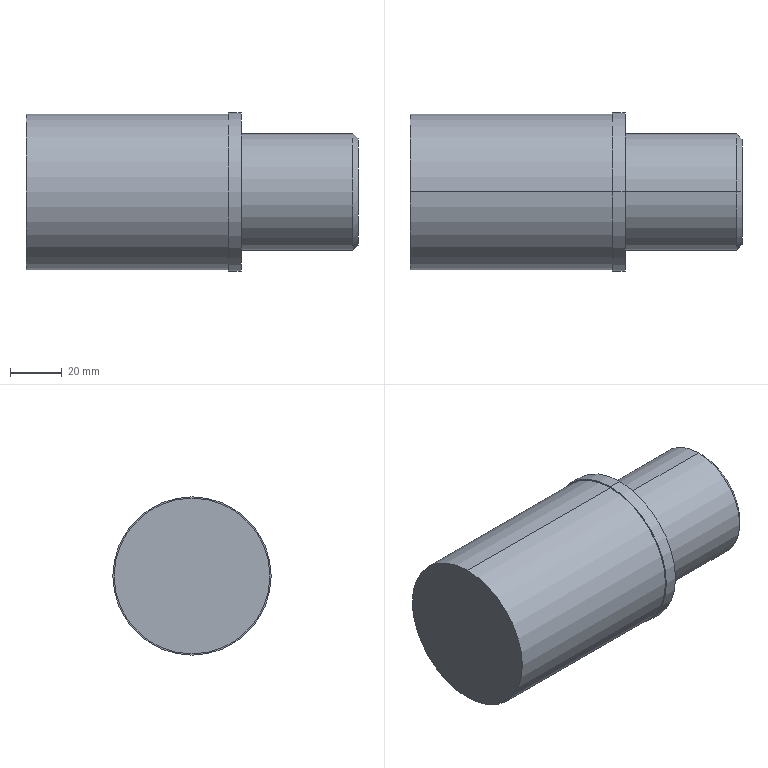Component | SolidWorks | YC1-250-03-01SliderAssembly-1_YC1-250-03-27BalancerConnectingPin-1 | 1 solid | 16 faces | box 128 x 61 x 61 mm | volume 305264 mm3 | cylinder 8 | cone 4 | plane 4 | commonest cylinder face diameters 60 x2 61 x2 45 x2 8.5 x2 | material Plain Carbon Steel
STEP:
#1=COLOUR_RGB('',0.7922,0.8196,0.9333);
#2=FILL_AREA_STYLE_COLOUR('',#1);
#3=FILL_AREA_STYLE('',(#2));
#4=SURFACE_STYLE_FILL_AREA(#3);
#5=SURFACE_SIDE_STYLE('',(#4));
#6=SURFACE_STYLE_USAGE(.BOTH.,#5);
#7=PRESENTATION_STYLE_ASSIGNMENT((#6));
#8=CARTESIAN_POINT('',(-16.732,110.632,1.181));
#9=VERTEX_POINT('',#8);
#10=CARTESIAN_POINT('',(-16.732,110.632,-1.181));
#11=VERTEX_POINT('',#10);
#12=CARTESIAN_POINT('',(-16.732,110.632,-0.));
#13=DIRECTION('',(-1.,0.,0.));
#14=DIRECTION('',(0.,0.,1.));
#15=AXIS2_PLACEMENT_3D('',#12,#13,#14);
#16=CIRCLE('',#15,1.181);
#17=EDGE_CURVE('',#9,#11,#16,.T.);
#18=ORIENTED_EDGE('',*,*,#17,.T.);
#19=CARTESIAN_POINT('',(-19.803,110.632,-1.181));
#20=VERTEX_POINT('',#19);
#21=CARTESIAN_POINT('',(-19.803,110.632,-1.181));
#22=DIRECTION('',(-1.,0.,0.));
#23=VECTOR('',#22,39.37);
#24=LINE('',#21,#23);
#25=EDGE_CURVE('',#11,#20,#24,.T.);
#26=ORIENTED_EDGE('',*,*,#25,.T.);
#27=CARTESIAN_POINT('',(-19.803,110.632,1.181));
#28=VERTEX_POINT('',#27);
#29=CARTESIAN_POINT('',(-19.803,110.632,-0.));
#30=DIRECTION('',(1.,0.,0.));
#31=DIRECTION('',(0.,0.,1.));
#32=AXIS2_PLACEMENT_3D('',#29,#30,#31);
#33=CIRCLE('',#32,1.181);
#34=EDGE_CURVE('',#20,#28,#33,.T.);
#35=ORIENTED_EDGE('',*,*,#34,.T.);
#36=CARTESIAN_POINT('',(-19.803,110.632,1.181));
#37=DIRECTION('',(-1.,0.,0.));
#38=VECTOR('',#37,39.37);
#39=LINE('',#36,#38);
#40=EDGE_CURVE('',#9,#28,#39,.T.);
#41=ORIENTED_EDGE('',*,*,#40,.F.);
#42=EDGE_LOOP('',(#18,#26,#35,#41));
#43=FACE_OUTER_BOUND('',#42,.T.);
#44=CARTESIAN_POINT('',(-19.803,110.632,-0.));
#45=DIRECTION('',(-1.,0.,0.));
#46=DIRECTION('',(0.,0.,1.));
#47=AXIS2_PLACEMENT_3D('',#44,#45,#46);
#48=CYLINDRICAL_SURFACE('',#47,1.181);
#49=ADVANCED_FACE('',(#43),#48,.T.);
#50=CARTESIAN_POINT('',(-16.535,110.632,1.201));
#51=VERTEX_POINT('',#50);
#52=CARTESIAN_POINT('',(-16.535,110.632,-1.201));
#53=VERTEX_POINT('',#52);
#54=CARTESIAN_POINT('',(-16.535,110.632,-0.));
#55=DIRECTION('',(-1.,0.,0.));
#56=DIRECTION('',(0.,0.,1.));
#57=AXIS2_PLACEMENT_3D('',#54,#55,#56);
#58=CIRCLE('',#57,1.201);
#59=EDGE_CURVE('',#51,#53,#58,.T.);
#60=ORIENTED_EDGE('',*,*,#59,.T.);
#61=CARTESIAN_POINT('',(-16.732,110.632,-1.201));
#62=VERTEX_POINT('',#61);
#63=CARTESIAN_POINT('',(-19.803,110.632,-1.201));
#64=DIRECTION('',(-1.,0.,0.));
#65=VECTOR('',#64,39.37);
#66=LINE('',#63,#65);
#67=EDGE_CURVE('',#53,#62,#66,.T.);
#68=ORIENTED_EDGE('',*,*,#67,.T.);
#69=CARTESIAN_POINT('',(-16.732,110.632,1.201));
#70=VERTEX_POINT('',#69);
#71=CARTESIAN_POINT('',(-16.732,110.632,-0.));
#72=DIRECTION('',(1.,0.,0.));
#73=DIRECTION('',(0.,0.,1.));
#74=AXIS2_PLACEMENT_3D('',#71,#72,#73);
#75=CIRCLE('',#74,1.201);
#76=EDGE_CURVE('',#62,#70,#75,.T.);
#77=ORIENTED_EDGE('',*,*,#76,.T.);
#78=CARTESIAN_POINT('',(-19.803,110.632,1.201));
#79=DIRECTION('',(-1.,0.,0.));
#80=VECTOR('',#79,39.37);
#81=LINE('',#78,#80);
#82=EDGE_CURVE('',#51,#70,#81,.T.);
#83=ORIENTED_EDGE('',*,*,#82,.F.);
#84=EDGE_LOOP('',(#60,#68,#77,#83));
#85=FACE_OUTER_BOUND('',#84,.T.);
#86=CARTESIAN_POINT('',(-19.803,110.632,-0.));
#87=DIRECTION('',(-1.,0.,0.));
#88=DIRECTION('',(0.,0.,1.));
#89=AXIS2_PLACEMENT_3D('',#86,#87,#88);
#90=CYLINDRICAL_SURFACE('',#89,1.201);
#91=ADVANCED_FACE('',(#85),#90,.T.);
#92=CARTESIAN_POINT('',(-14.843,110.632,0.8858));
#93=VERTEX_POINT('',#92);
#94=CARTESIAN_POINT('',(-14.843,110.632,-0.8858));
#95=VERTEX_POINT('',#94);
#96=CARTESIAN_POINT('',(-14.843,110.632,-0.));
#97=DIRECTION('',(-1.,0.,0.));
#98=DIRECTION('',(0.,0.,1.));
#99=AXIS2_PLACEMENT_3D('',#96,#97,#98);
#100=CIRCLE('',#99,0.8858);
#101=EDGE_CURVE('',#93,#95,#100,.T.);
#102=ORIENTED_EDGE('',*,*,#101,.T.);
#103=CARTESIAN_POINT('',(-16.535,110.632,-0.8858));
#104=VERTEX_POINT('',#103);
#105=CARTESIAN_POINT('',(-19.803,110.632,-0.8858));
#106=DIRECTION('',(-1.,0.,0.));
#107=VECTOR('',#106,39.37);
#108=LINE('',#105,#107);
#109=EDGE_CURVE('',#95,#104,#108,.T.);
#110=ORIENTED_EDGE('',*,*,#109,.T.);
#111=CARTESIAN_POINT('',(-16.535,110.632,0.8858));
#112=VERTEX_POINT('',#111);
#113=CARTESIAN_POINT('',(-16.535,110.632,-0.));
#114=DIRECTION('',(1.,0.,0.));
#115=DIRECTION('',(0.,0.,1.));
#116=AXIS2_PLACEMENT_3D('',#113,#114,#115);
#117=CIRCLE('',#116,0.8858);
#118=EDGE_CURVE('',#104,#112,#117,.T.);
#119=ORIENTED_EDGE('',*,*,#118,.T.);
#120=CARTESIAN_POINT('',(-19.803,110.632,0.8858));
#121=DIRECTION('',(-1.,0.,0.));
#122=VECTOR('',#121,39.37);
#123=LINE('',#120,#122);
#124=EDGE_CURVE('',#93,#112,#123,.T.);
#125=ORIENTED_EDGE('',*,*,#124,.F.);
#126=EDGE_LOOP('',(#102,#110,#119,#125));
#127=FACE_OUTER_BOUND('',#126,.T.);
#128=CARTESIAN_POINT('',(-19.803,110.632,-0.));
#129=DIRECTION('',(-1.,0.,0.));
#130=DIRECTION('',(0.,0.,1.));
#131=AXIS2_PLACEMENT_3D('',#128,#129,#130);
#132=CYLINDRICAL_SURFACE('',#131,0.8858);
#133=ADVANCED_FACE('',(#127),#132,.T.);
#134=CARTESIAN_POINT('',(-14.764,110.632,0.8071));
#135=VERTEX_POINT('',#134);
#136=CARTESIAN_POINT('',(-14.764,110.632,-0.8071));
#137=VERTEX_POINT('',#136);
#138=CARTESIAN_POINT('',(-14.764,110.632,-0.));
#139=DIRECTION('',(-1.,0.,0.));
#140=DIRECTION('',(0.,0.,1.));
#141=AXIS2_PLACEMENT_3D('',#138,#139,#140);
#142=CIRCLE('',#141,0.8071);
#143=EDGE_CURVE('',#135,#137,#142,.T.);
#144=ORIENTED_EDGE('',*,*,#143,.T.);
#145=CARTESIAN_POINT('',(-14.843,110.632,-0.8858));
#146=DIRECTION('',(-0.7071,0.,-0.7071));
#147=VECTOR('',#146,39.37);
#148=LINE('',#145,#147);
#149=EDGE_CURVE('',#137,#95,#148,.T.);
#150=ORIENTED_EDGE('',*,*,#149,.T.);
#151=ORIENTED_EDGE('',*,*,#101,.F.);
#152=CARTESIAN_POINT('',(-14.843,110.632,0.8858));
#153=DIRECTION('',(-0.7071,0.,0.7071));
#154=VECTOR('',#153,39.37);
#155=LINE('',#152,#154);
#156=EDGE_CURVE('',#135,#93,#155,.T.);
#157=ORIENTED_EDGE('',*,*,#156,.F.);
#158=EDGE_LOOP('',(#144,#150,#151,#157));
#159=FACE_OUTER_BOUND('',#158,.T.);
#160=CARTESIAN_POINT('',(-14.843,110.632,-0.));
#161=DIRECTION('',(-1.,0.,0.));
#162=DIRECTION('',(0.,0.,1.));
#163=AXIS2_PLACEMENT_3D('',#160,#161,#162);
#164=CONICAL_SURFACE('',#163,0.8858,0.7854);
#165=ADVANCED_FACE('',(#159),#164,.T.);
#166=CARTESIAN_POINT('',(-15.551,110.632,0.1673));
#167=VERTEX_POINT('',#166);
#168=CARTESIAN_POINT('',(-15.551,110.632,-0.1673));
#169=VERTEX_POINT('',#168);
#170=CARTESIAN_POINT('',(-15.551,110.632,-0.));
#171=DIRECTION('',(1.,0.,0.));
#172=DIRECTION('',(0.,0.,-1.));
#173=AXIS2_PLACEMENT_3D('',#170,#171,#172);
#174=CIRCLE('',#173,0.1673);
#175=EDGE_CURVE('',#167,#169,#174,.T.);
#176=ORIENTED_EDGE('',*,*,#175,.F.);
#177=CARTESIAN_POINT('',(-14.764,110.632,0.1673));
#178=VERTEX_POINT('',#177);
#179=CARTESIAN_POINT('',(-14.764,110.632,0.1673));
#180=DIRECTION('',(1.,0.,0.));
#181=VECTOR('',#180,39.37);
#182=LINE('',#179,#181);
#183=EDGE_CURVE('',#167,#178,#182,.T.);
#184=ORIENTED_EDGE('',*,*,#183,.T.);
#185=CARTESIAN_POINT('',(-14.764,110.632,-0.1673));
#186=VERTEX_POINT('',#185);
#187=CARTESIAN_POINT('',(-14.764,110.632,-0.));
#188=DIRECTION('',(1.,0.,0.));
#189=DIRECTION('',(0.,0.,-1.));
#190=AXIS2_PLACEMENT_3D('',#187,#188,#189);
#191=CIRCLE('',#190,0.1673);
#192=EDGE_CURVE('',#178,#186,#191,.T.);
#193=ORIENTED_EDGE('',*,*,#192,.T.);
#194=CARTESIAN_POINT('',(-14.764,110.632,-0.1673));
#195=DIRECTION('',(1.,0.,0.));
#196=VECTOR('',#195,39.37);
#197=LINE('',#194,#196);
#198=EDGE_CURVE('',#169,#186,#197,.T.);
#199=ORIENTED_EDGE('',*,*,#198,.F.);
#200=EDGE_LOOP('',(#176,#184,#193,#199));
#201=FACE_OUTER_BOUND('',#200,.T.);
#202=CARTESIAN_POINT('',(-14.764,110.632,-0.));
#203=DIRECTION('',(1.,0.,0.));
#204=DIRECTION('',(0.,0.,-1.));
#205=AXIS2_PLACEMENT_3D('',#202,#203,#204);
#206=CYLINDRICAL_SURFACE('',#205,0.1673);
#207=ADVANCED_FACE('',(#201),#206,.F.);
#208=CARTESIAN_POINT('',(-15.652,110.632,-0.));
#209=VERTEX_POINT('',#208);
#210=CARTESIAN_POINT('',(-15.551,110.632,-0.1673));
#211=DIRECTION('',(0.515,0.,-0.8572));
#212=VECTOR('',#211,39.37);
#213=LINE('',#210,#212);
#214=EDGE_CURVE('',#209,#169,#213,.T.);
#215=ORIENTED_EDGE('',*,*,#214,.F.);
#216=CARTESIAN_POINT('',(-15.551,110.632,0.1673));
#217=DIRECTION('',(0.515,0.,0.8572));
#218=VECTOR('',#217,39.37);
#219=LINE('',#216,#218);
#220=EDGE_CURVE('',#209,#167,#219,.T.);
#221=ORIENTED_EDGE('',*,*,#220,.T.);
#222=ORIENTED_EDGE('',*,*,#175,.T.);
#223=EDGE_LOOP('',(#215,#221,#222));
#224=FACE_OUTER_BOUND('',#223,.T.);
#225=CARTESIAN_POINT('',(-15.551,110.632,-0.));
#226=DIRECTION('',(1.,0.,0.));
#227=DIRECTION('',(0.,0.,-1.));
#228=AXIS2_PLACEMENT_3D('',#225,#226,#227);
#229=CONICAL_SURFACE('',#228,0.1673,1.03);
#230=ADVANCED_FACE('',(#224),#229,.F.);
#231=ORIENTED_EDGE('',*,*,#25,.F.);
#232=CARTESIAN_POINT('',(-16.732,110.632,-0.));
#233=DIRECTION('',(-1.,0.,0.));
#234=DIRECTION('',(0.,0.,1.));
#235=AXIS2_PLACEMENT_3D('',#232,#233,#234);
#236=CIRCLE('',#235,1.181);
#237=EDGE_CURVE('',#11,#9,#236,.T.);
#238=ORIENTED_EDGE('',*,*,#237,.T.);
#239=ORIENTED_EDGE('',*,*,#40,.T.);
#240=CARTESIAN_POINT('',(-19.803,110.632,-0.));
#241=DIRECTION('',(1.,0.,0.));
#242=DIRECTION('',(0.,0.,1.));
#243=AXIS2_PLACEMENT_3D('',#240,#241,#242);
#244=CIRCLE('',#243,1.181);
#245=EDGE_CURVE('',#28,#20,#244,.T.);
#246=ORIENTED_EDGE('',*,*,#245,.T.);
#247=EDGE_LOOP('',(#231,#238,#239,#246));
#248=FACE_OUTER_BOUND('',#247,.T.);
#249=CARTESIAN_POINT('',(-19.803,110.632,-0.));
#250=DIRECTION('',(-1.,0.,0.));
#251=DIRECTION('',(0.,0.,1.));
#252=AXIS2_PLACEMENT_3D('',#249,#250,#251);
#253=CYLINDRICAL_SURFACE('',#252,1.181);
#254=ADVANCED_FACE('',(#248),#253,.T.);
#255=ORIENTED_EDGE('',*,*,#245,.F.);
#256=ORIENTED_EDGE('',*,*,#34,.F.);
#257=EDGE_LOOP('',(#255,#256));
#258=FACE_OUTER_BOUND('',#257,.T.);
#259=CARTESIAN_POINT('',(-19.803,110.632,-0.));
#260=DIRECTION('',(1.,0.,0.));
#261=DIRECTION('',(0.,0.,-1.));
#262=AXIS2_PLACEMENT_3D('',#259,#260,#261);
#263=PLANE('',#262);
#264=ADVANCED_FACE('',(#258),#263,.F.);
#265=CARTESIAN_POINT('',(-16.732,110.632,-0.));
#266=DIRECTION('',(1.,0.,0.));
#267=DIRECTION('',(0.,0.,1.));
#268=AXIS2_PLACEMENT_3D('',#265,#266,#267);
#269=CIRCLE('',#268,1.201);
#270=EDGE_CURVE('',#70,#62,#269,.T.);
#271=ORIENTED_EDGE('',*,*,#270,.F.);
#272=ORIENTED_EDGE('',*,*,#76,.F.);
#273=EDGE_LOOP('',(#271,#272));
#274=FACE_OUTER_BOUND('',#273,.T.);
#275=ORIENTED_EDGE('',*,*,#17,.F.);
#276=ORIENTED_EDGE('',*,*,#237,.F.);
#277=EDGE_LOOP('',(#275,#276));
#278=FACE_BOUND('',#277,.T.);
#279=CARTESIAN_POINT('',(-16.732,111.813,-0.));
#280=DIRECTION('',(1.,0.,0.));
#281=DIRECTION('',(0.,0.,-1.));
#282=AXIS2_PLACEMENT_3D('',#279,#280,#281);
#283=PLANE('',#282);
#284=ADVANCED_FACE('',(#274,#278),#283,.F.);
#285=ORIENTED_EDGE('',*,*,#67,.F.);
#286=CARTESIAN_POINT('',(-16.535,110.632,-0.));
#287=DIRECTION('',(-1.,0.,0.));
#288=DIRECTION('',(0.,0.,1.));
#289=AXIS2_PLACEMENT_3D('',#286,#287,#288);
#290=CIRCLE('',#289,1.201);
#291=EDGE_CURVE('',#53,#51,#290,.T.);
#292=ORIENTED_EDGE('',*,*,#291,.T.);
#293=ORIENTED_EDGE('',*,*,#82,.T.);
#294=ORIENTED_EDGE('',*,*,#270,.T.);
#295=EDGE_LOOP('',(#285,#292,#293,#294));
#296=FACE_OUTER_BOUND('',#295,.T.);
#297=CARTESIAN_POINT('',(-19.803,110.632,-0.));
#298=DIRECTION('',(-1.,0.,0.));
#299=DIRECTION('',(0.,0.,1.));
#300=AXIS2_PLACEMENT_3D('',#297,#298,#299);
#301=CYLINDRICAL_SURFACE('',#300,1.201);
#302=ADVANCED_FACE('',(#296),#301,.T.);
#303=CARTESIAN_POINT('',(-16.535,110.632,-0.));
#304=DIRECTION('',(1.,0.,0.));
#305=DIRECTION('',(0.,0.,1.));
#306=AXIS2_PLACEMENT_3D('',#303,#304,#305);
#307=CIRCLE('',#306,0.8858);
#308=EDGE_CURVE('',#112,#104,#307,.T.);
#309=ORIENTED_EDGE('',*,*,#308,.F.);
#310=ORIENTED_EDGE('',*,*,#118,.F.);
#311=EDGE_LOOP('',(#309,#310));
#312=FACE_BOUND('',#311,.T.);
#313=ORIENTED_EDGE('',*,*,#59,.F.);
#314=ORIENTED_EDGE('',*,*,#291,.F.);
#315=EDGE_LOOP('',(#313,#314));
#316=FACE_OUTER_BOUND('',#315,.T.);
#317=CARTESIAN_POINT('',(-16.535,111.833,-0.));
#318=DIRECTION('',(-1.,0.,0.));
#319=DIRECTION('',(0.,0.,1.));
#320=AXIS2_PLACEMENT_3D('',#317,#318,#319);
#321=PLANE('',#320);
#322=ADVANCED_FACE('',(#312,#316),#321,.F.);
#323=ORIENTED_EDGE('',*,*,#109,.F.);
#324=CARTESIAN_POINT('',(-14.843,110.632,-0.));
#325=DIRECTION('',(-1.,0.,0.));
#326=DIRECTION('',(0.,0.,1.));
#327=AXIS2_PLACEMENT_3D('',#324,#325,#326);
#328=CIRCLE('',#327,0.8858);
#329=EDGE_CURVE('',#95,#93,#328,.T.);
#330=ORIENTED_EDGE('',*,*,#329,.T.);
#331=ORIENTED_EDGE('',*,*,#124,.T.);
#332=ORIENTED_EDGE('',*,*,#308,.T.);
#333=EDGE_LOOP('',(#323,#330,#331,#332));
#334=FACE_OUTER_BOUND('',#333,.T.);
#335=CARTESIAN_POINT('',(-19.803,110.632,-0.));
#336=DIRECTION('',(-1.,0.,0.));
#337=DIRECTION('',(0.,0.,1.));
#338=AXIS2_PLACEMENT_3D('',#335,#336,#337);
#339=CYLINDRICAL_SURFACE('',#338,0.8858);
#340=ADVANCED_FACE('',(#334),#339,.T.);
#341=ORIENTED_EDGE('',*,*,#149,.F.);
#342=CARTESIAN_POINT('',(-14.764,110.632,-0.));
#343=DIRECTION('',(-1.,0.,0.));
#344=DIRECTION('',(0.,0.,1.));
#345=AXIS2_PLACEMENT_3D('',#342,#343,#344);
#346=CIRCLE('',#345,0.8071);
#347=EDGE_CURVE('',#137,#135,#346,.T.);
#348=ORIENTED_EDGE('',*,*,#347,.T.);
#349=ORIENTED_EDGE('',*,*,#156,.T.);
#350=ORIENTED_EDGE('',*,*,#329,.F.);
#351=EDGE_LOOP('',(#341,#348,#349,#350));
#352=FACE_OUTER_BOUND('',#351,.T.);
#353=CARTESIAN_POINT('',(-14.843,110.632,-0.));
#354=DIRECTION('',(-1.,0.,0.));
#355=DIRECTION('',(0.,0.,1.));
#356=AXIS2_PLACEMENT_3D('',#353,#354,#355);
#357=CONICAL_SURFACE('',#356,0.8858,0.7854);
#358=ADVANCED_FACE('',(#352),#357,.T.);
#359=ORIENTED_EDGE('',*,*,#143,.F.);
#360=ORIENTED_EDGE('',*,*,#347,.F.);
#361=EDGE_LOOP('',(#359,#360));
#362=FACE_OUTER_BOUND('',#361,.T.);
#363=CARTESIAN_POINT('',(-14.764,110.632,-0.));
#364=DIRECTION('',(1.,0.,0.));
#365=DIRECTION('',(0.,0.,-1.));
#366=AXIS2_PLACEMENT_3D('',#363,#364,#365);
#367=CIRCLE('',#366,0.1673);
#368=EDGE_CURVE('',#186,#178,#367,.T.);
#369=ORIENTED_EDGE('',*,*,#368,.F.);
#370=ORIENTED_EDGE('',*,*,#192,.F.);
#371=EDGE_LOOP('',(#369,#370));
#372=FACE_BOUND('',#371,.T.);
#373=CARTESIAN_POINT('',(-14.764,111.518,-0.));
#374=DIRECTION('',(-1.,0.,0.));
#375=DIRECTION('',(0.,0.,1.));
#376=AXIS2_PLACEMENT_3D('',#373,#374,#375);
#377=PLANE('',#376);
#378=ADVANCED_FACE('',(#362,#372),#377,.F.);
#379=ORIENTED_EDGE('',*,*,#183,.F.);
#380=CARTESIAN_POINT('',(-15.551,110.632,-0.));
#381=DIRECTION('',(1.,0.,0.));
#382=DIRECTION('',(0.,0.,-1.));
#383=AXIS2_PLACEMENT_3D('',#380,#381,#382);
#384=CIRCLE('',#383,0.1673);
#385=EDGE_CURVE('',#169,#167,#384,.T.);
#386=ORIENTED_EDGE('',*,*,#385,.F.);
#387=ORIENTED_EDGE('',*,*,#198,.T.);
#388=ORIENTED_EDGE('',*,*,#368,.T.);
#389=EDGE_LOOP('',(#379,#386,#387,#388));
#390=FACE_OUTER_BOUND('',#389,.T.);
#391=CARTESIAN_POINT('',(-14.764,110.632,-0.));
#392=DIRECTION('',(1.,0.,0.));
#393=DIRECTION('',(0.,0.,-1.));
#394=AXIS2_PLACEMENT_3D('',#391,#392,#393);
#395=CYLINDRICAL_SURFACE('',#394,0.1673);
#396=ADVANCED_FACE('',(#390),#395,.F.);
#397=ORIENTED_EDGE('',*,*,#220,.F.);
#398=ORIENTED_EDGE('',*,*,#214,.T.);
#399=ORIENTED_EDGE('',*,*,#385,.T.);
#400=EDGE_LOOP('',(#397,#398,#399));
#401=FACE_OUTER_BOUND('',#400,.T.);
#402=CARTESIAN_POINT('',(-15.551,110.632,-0.));
#403=DIRECTION('',(1.,0.,0.));
#404=DIRECTION('',(0.,0.,-1.));
#405=AXIS2_PLACEMENT_3D('',#402,#403,#404);
#406=CONICAL_SURFACE('',#405,0.1673,1.03);
#407=ADVANCED_FACE('',(#401),#406,.F.);
#408=CLOSED_SHELL('',(#49,#91,#133,#165,#207,#230,#254,#264,#284,#302,#322,#340,#358,#378,#396,#407));
#409=MANIFOLD_SOLID_BREP('',#408);
#410=STYLED_ITEM('',(#7),#409);
#411=(LENGTH_UNIT()NAMED_UNIT(*)SI_UNIT($,.METRE.));
#412=LENGTH_MEASURE_WITH_UNIT(LENGTH_MEASURE(0.0254),#411);
#413=DIMENSIONAL_EXPONENTS(1.,0.,0.,0.,0.,0.,0.);
#414=(CONVERSION_BASED_UNIT('',#412)LENGTH_UNIT()NAMED_UNIT(#413));
#415=UNCERTAINTY_MEASURE_WITH_UNIT(LENGTH_MEASURE(0.00001),#414,'','');
#416=(NAMED_UNIT(*)PLANE_ANGLE_UNIT()SI_UNIT($,.RADIAN.));
#417=(NAMED_UNIT(*)SI_UNIT($,.STERADIAN.)SOLID_ANGLE_UNIT());
#418=(GEOMETRIC_REPRESENTATION_CONTEXT(3)GLOBAL_UNCERTAINTY_ASSIGNED_CONTEXT((#415))GLOBAL_UNIT_ASSIGNED_CONTEXT((#414,#416,#417))REPRESENTATION_CONTEXT('',''));
#419=MECHANICAL_DESIGN_GEOMETRIC_PRESENTATION_REPRESENTATION('',(#410),#418);
#420=CARTESIAN_POINT('',(0.,0.,0.));
#421=DIRECTION('',(0.,0.,1.));
#422=DIRECTION('',(1.,0.,0.));
#423=AXIS2_PLACEMENT_3D('',#420,#421,#422);
#424=(LENGTH_UNIT()NAMED_UNIT(*)SI_UNIT($,.METRE.));
#425=LENGTH_MEASURE_WITH_UNIT(LENGTH_MEASURE(0.0254),#424);
#426=DIMENSIONAL_EXPONENTS(1.,0.,0.,0.,0.,0.,0.);
#427=(CONVERSION_BASED_UNIT('',#425)LENGTH_UNIT()NAMED_UNIT(#426));
#428=UNCERTAINTY_MEASURE_WITH_UNIT(LENGTH_MEASURE(0.00001),#427,'','');
#429=(NAMED_UNIT(*)PLANE_ANGLE_UNIT()SI_UNIT($,.RADIAN.));
#430=(NAMED_UNIT(*)SI_UNIT($,.STERADIAN.)SOLID_ANGLE_UNIT());
#431=(GEOMETRIC_REPRESENTATION_CONTEXT(3)GLOBAL_UNCERTAINTY_ASSIGNED_CONTEXT((#428))GLOBAL_UNIT_ASSIGNED_CONTEXT((#427,#429,#430))REPRESENTATION_CONTEXT('',''));
#432=ADVANCED_BREP_SHAPE_REPRESENTATION('',(#409,#423),#431);
#433=PRESENTATION_LAYER_ASSIGNMENT('','',(#410));